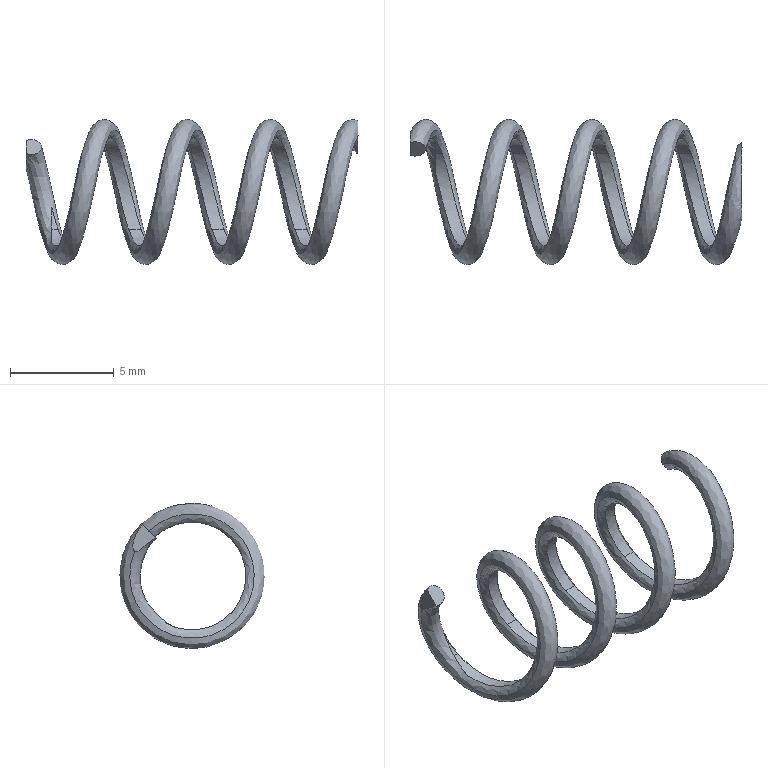Component | SolidWorks | VUM5-30-2 | 1 solid | 16 faces | volume 56 mm3 | cylinder 9 | plane 5 | spline 2 | commonest cylinder face diameters 5.2 x9